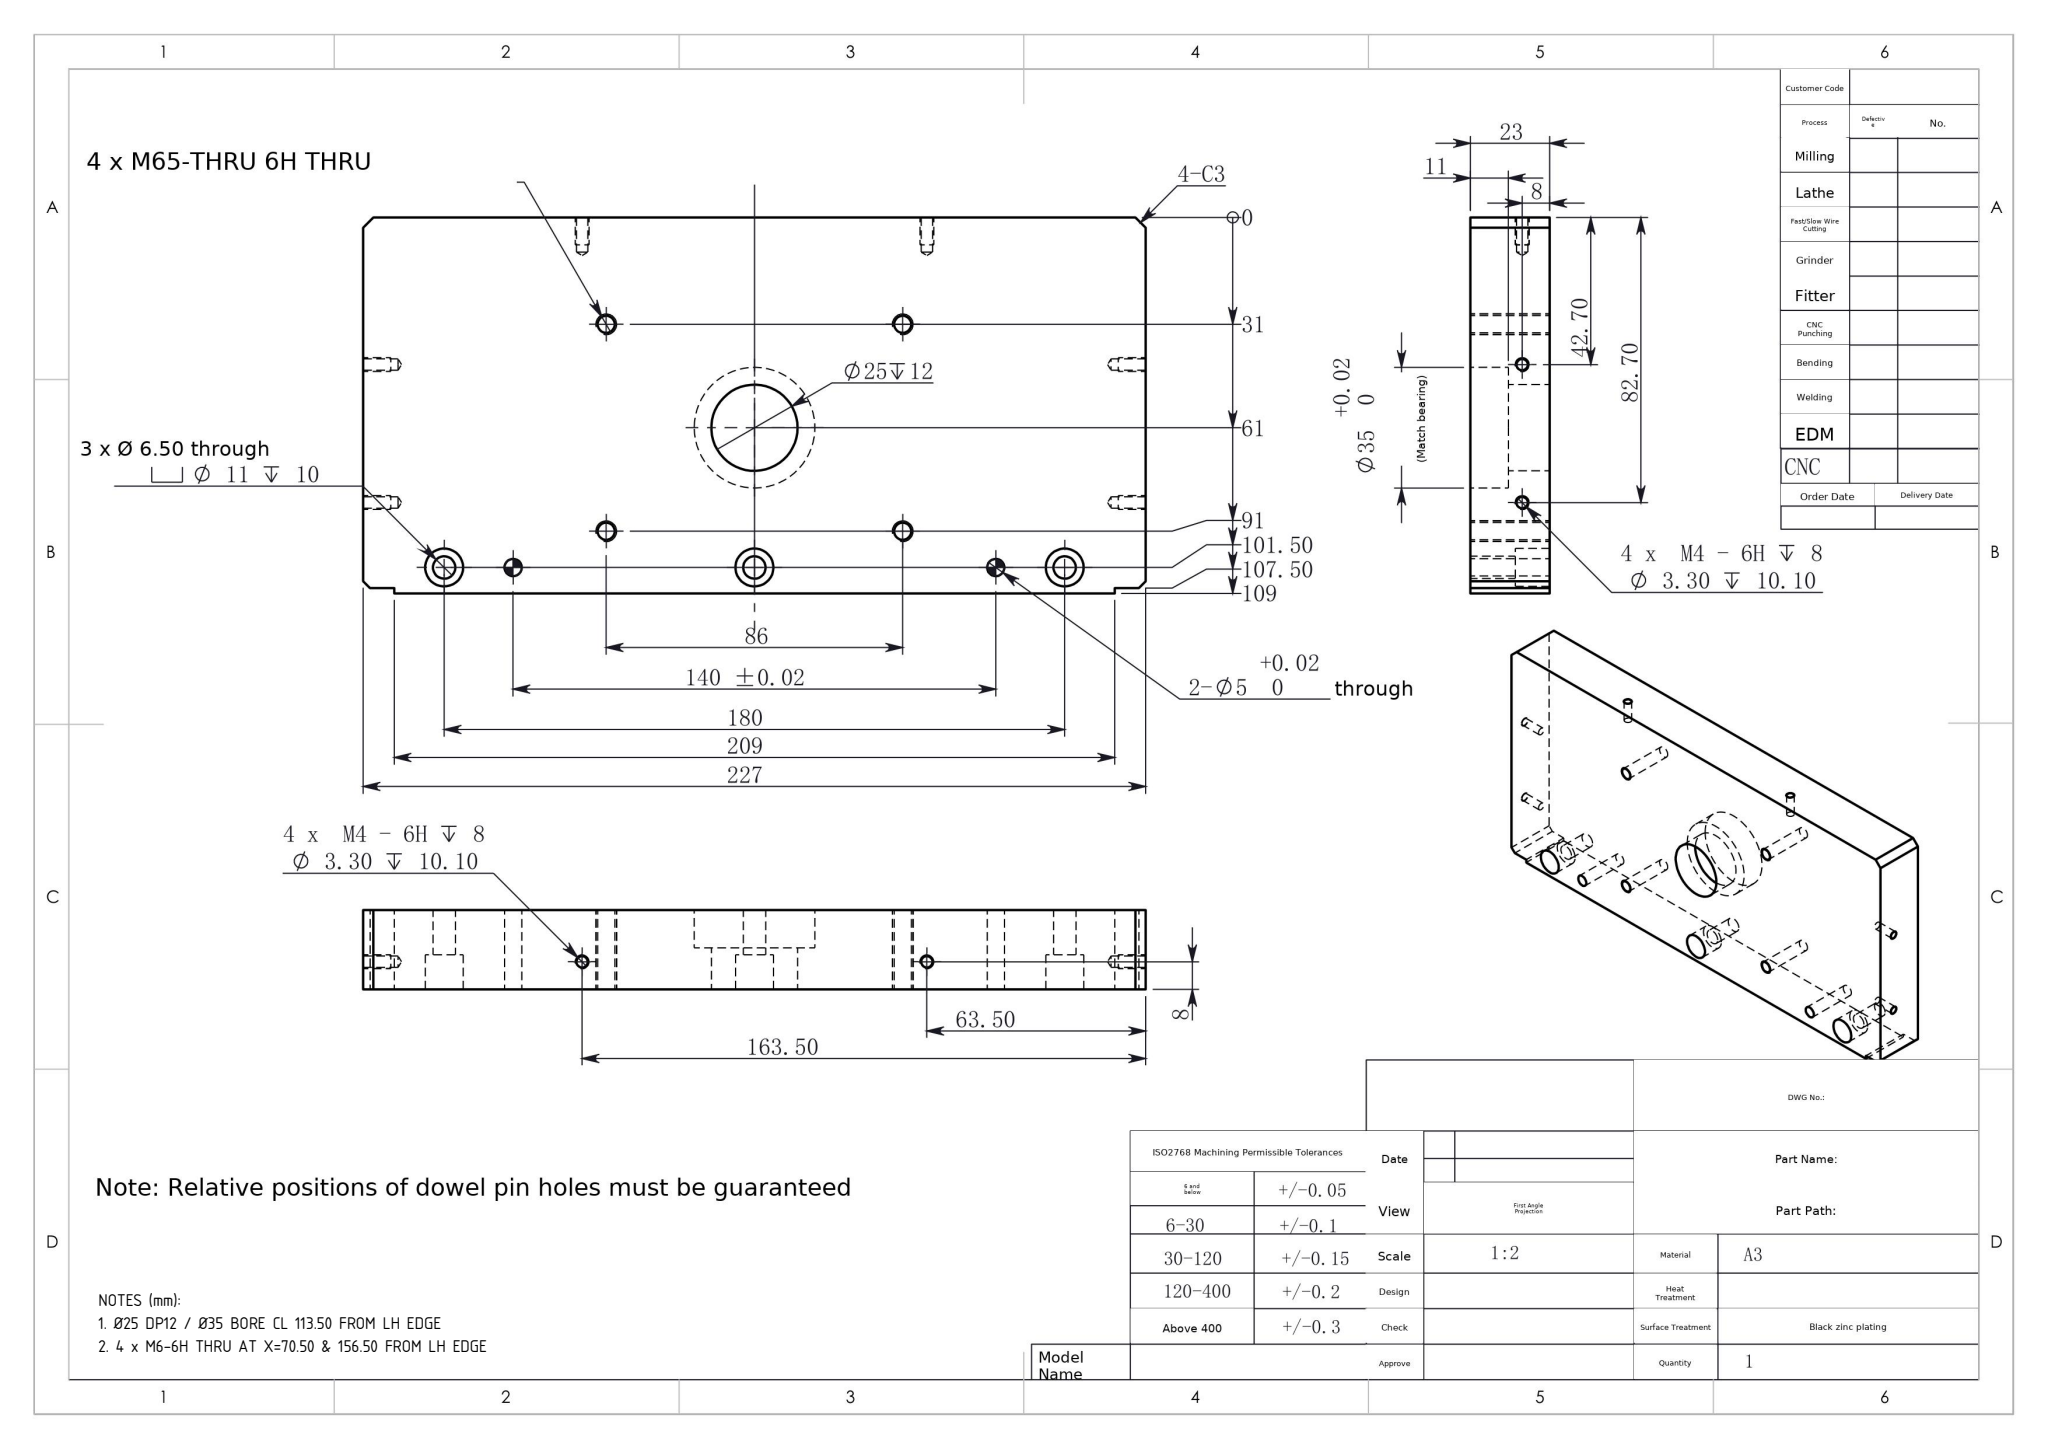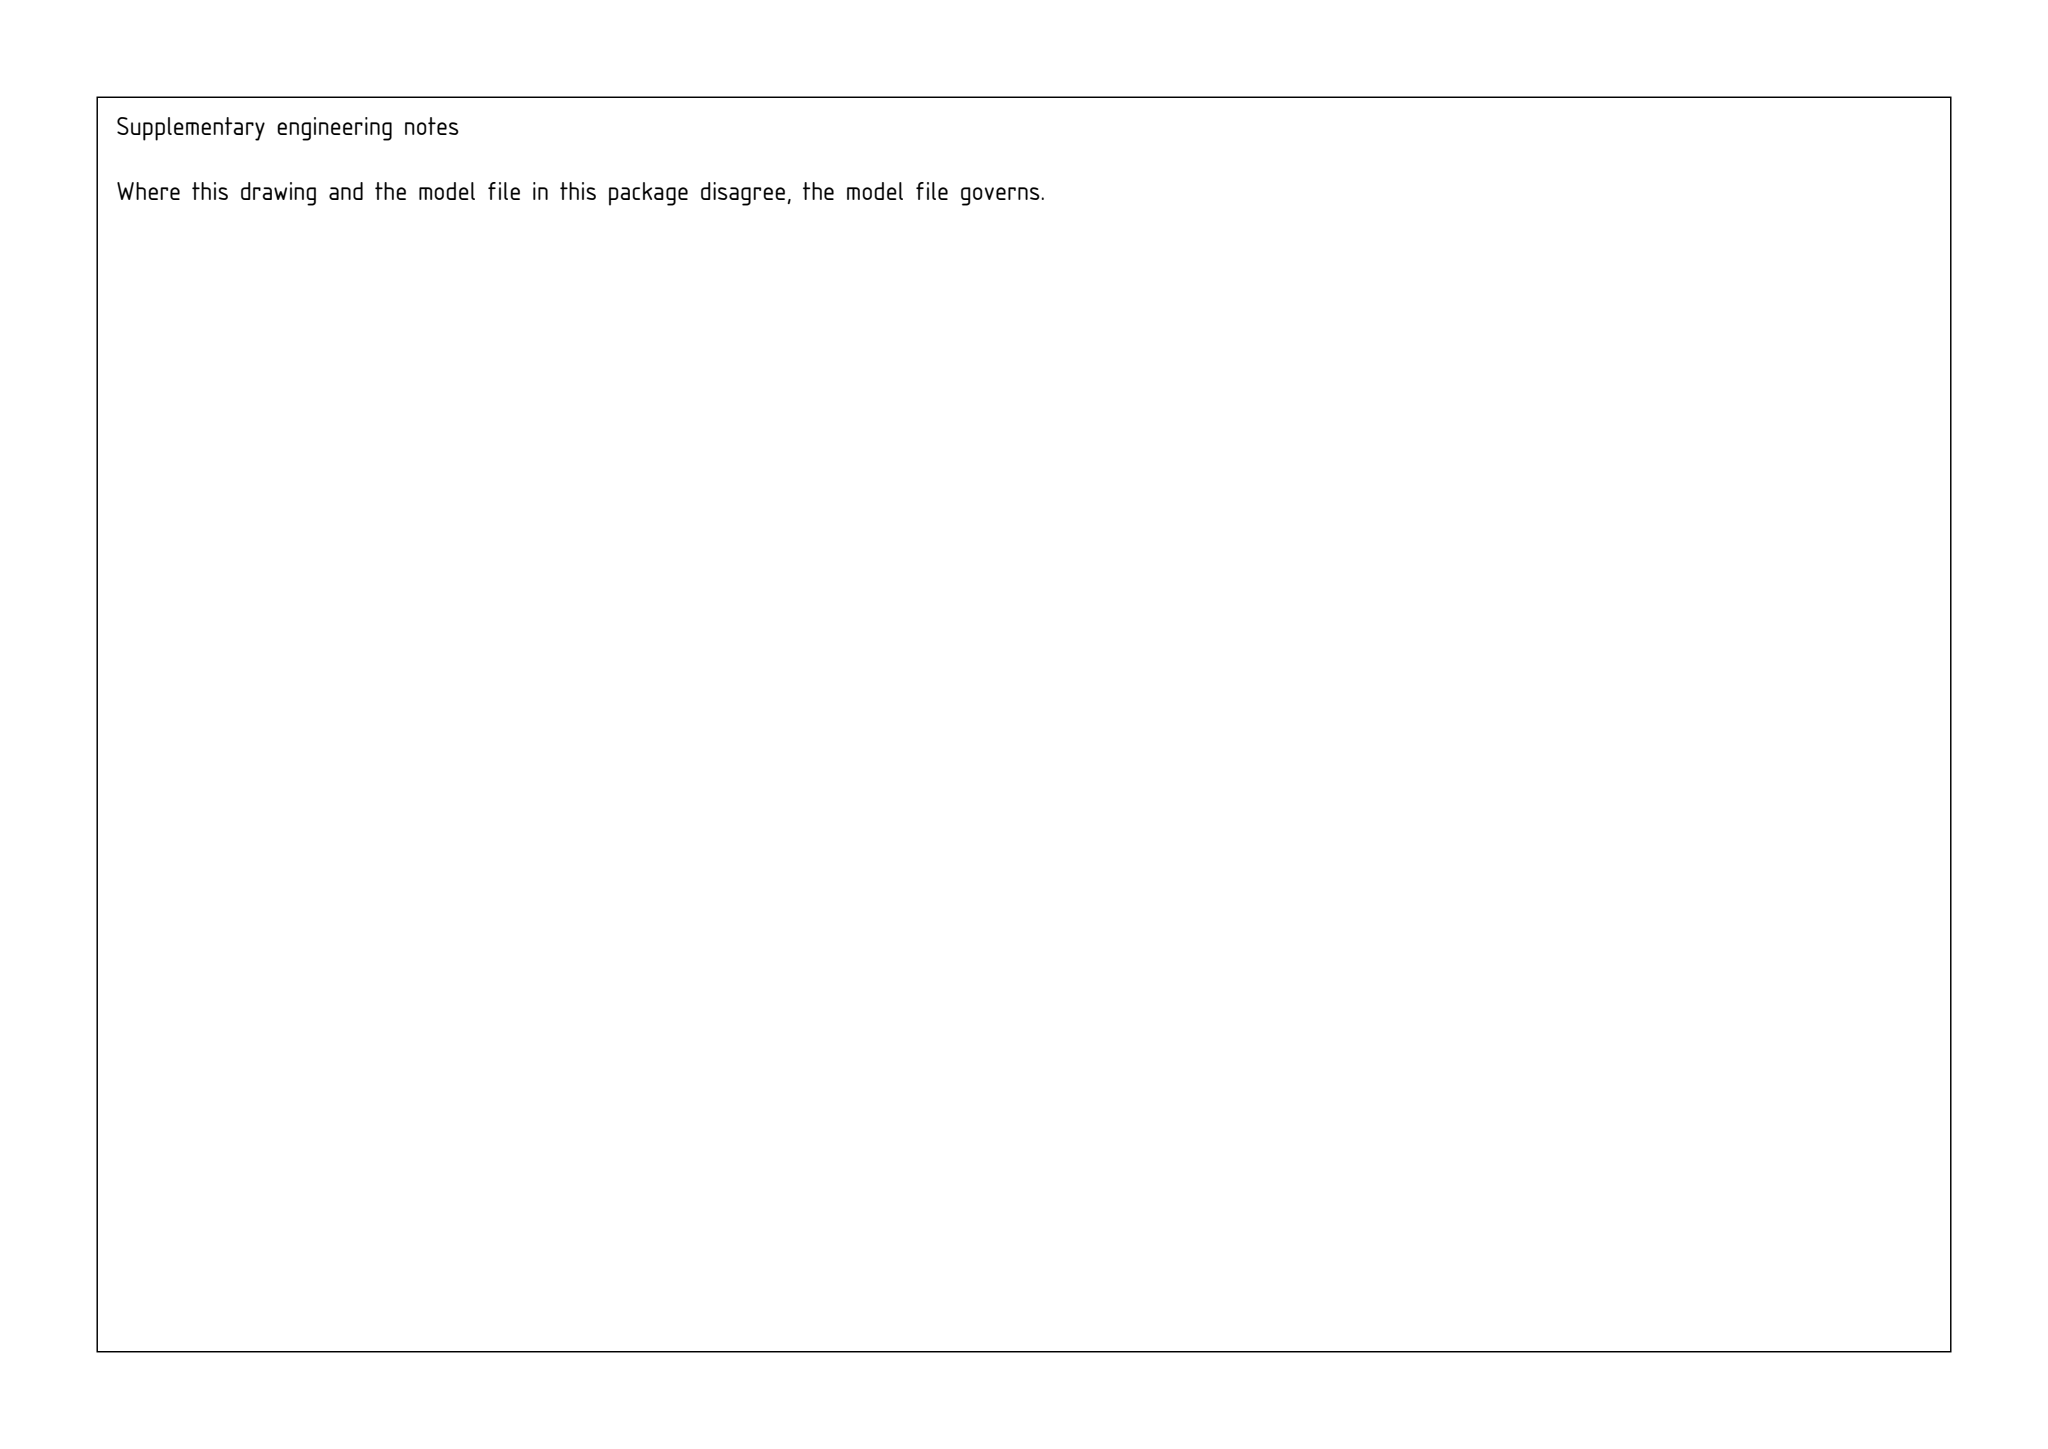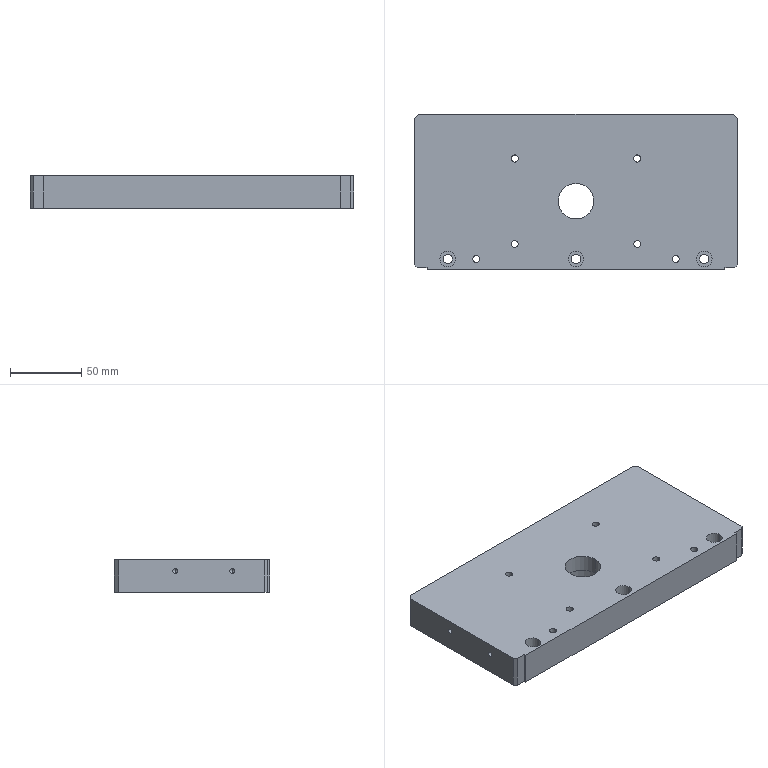Part | SolidWorks | mm | 1 solid | 70 faces | box 227 x 109 x 23 mm | volume 544305 mm3 | cylinder 40 | plane 18 | cone 12 | commonest cylinder face diameters 3.3 x12 5 x12 11 x6 6.5 x6 35 x2 25 x2
Drawing notes:
Ø25 DP12 / Ø35 BORE CL 113.50 FROM LH EDGE | from the solid: Ø25 L12 and Ø35 L11 z-cylinders at (113.5,48.0); bbox X=227, so CL = mid-width
4 x M6-6H THRU AT X=70.50 & 156.50 FROM LH EDGE | from the solid: Ø5.0 z-holes thru 23 at (70.5,18),(70.5,78),(156.5,18),(156.5,78); Ø5 = M6 tap drill
build123d program:
from build123d import *

# Parameters (mm, degrees)
SKETCH4_W                                          = 227
SKETCH4_H                                          = 109
SKETCH4_R                                          = 12.5
SKETCH4_R_2                                        = 2.5
BOSS_EXTRUDE1_DEPTH                                = 23
CHAMFER1_SIZE                                      = 3
HOLE_SIZE_ACCORDING_TO_TYPE_1_OF_HEXAG_D           = 6.5
HOLE_SIZE_ACCORDING_TO_TYPE_1_OF_HEXAG_CBORE_D     = 11
HOLE_SIZE_ACCORDING_TO_TYPE_1_OF_HEXAG_CBORE_DEPTH = 10
M6_TAPPED_HOLE1_D                                  = 5
M4_TAPPED_HOLE2_AT_2_COUNT                         = 2
M4_TAPPED_HOLE2_AT_2_PITCH                         = 40
M4_TAPPED_HOLE3_D                                  = 3.3
M4_TAPPED_HOLE3_DEPTH                              = 10.1
M4_TAPPED_HOLE3_TIP                                = 0.9914
SKETCH17_W                                         = 9
SKETCH17_H                                         = 1.5
CUT_EXTRUDE2_DEPTH                                 = 128.99
CHAMFER2_SIZE                                      = 2
SKETCH10_R                                         = 17.5
CUT_EXTRUDE3_DEPTH                                 = 11


with BuildPart() as part:
    # Sketch4 → Boss-Extrude1 (new body)
    with BuildSketch(Plane.XY):
        Rectangle(SKETCH4_W, SKETCH4_H)
        with Locations((0, -6.5)):
            Circle(SKETCH4_R, mode=Mode.SUBTRACT)
        with Locations((-70, -47)):
            Circle(SKETCH4_R_2, mode=Mode.SUBTRACT)
        with Locations(Location((70, -47, 0), (0, 0, 180))):
            Circle(SKETCH4_R_2, mode=Mode.SUBTRACT)
    extrude(amount=BOSS_EXTRUDE1_DEPTH)

    # Chamfer1
    chamfer1_edges = [part.edges().sort_by_distance(p)[0] for p in [
        (-113.5, 54.5, 11.5),
        (113.5, 54.5, 11.5),
    ]]
    chamfer(chamfer1_edges, length=CHAMFER1_SIZE)

    # Hole Size _According to_ Type 1 of Hexag (through all)
    with Locations(Plane.XY.offset(23)):
        with Locations((90, -47), (-90, -47), (0, -47)):
            CounterBoreHole(HOLE_SIZE_ACCORDING_TO_TYPE_1_OF_HEXAG_D / 2, HOLE_SIZE_ACCORDING_TO_TYPE_1_OF_HEXAG_CBORE_D / 2, HOLE_SIZE_ACCORDING_TO_TYPE_1_OF_HEXAG_CBORE_DEPTH)

    # M6 Tapped Hole1 (through all)
    with Locations(Plane.XY.offset(23)):
        with Locations((-43, -36.5), (-43, 23.5), (43, 23.5), (43, -36.5)):
            Hole(M6_TAPPED_HOLE1_D / 2)

    # Sketch14 → M4 Tapped Hole2 (revolve, cut)
    with BuildSketch(Plane(origin=(-113.5, -28.2, 15), x_dir=(0, 0, 1), z_dir=(0, 1, 0))):
        Polygon((0, 0), (0, 11.091), (1.65, 10.1), (1.65, 0), align=None)
    m4_tapped_hole2 = revolve(axis=Axis((-119.85, -28.2, 15), (1, 0, 0)), mode=Mode.SUBTRACT)

    # M4 Tapped Hole2 at 2: M4 Tapped Hole2 ×2
    with Locations(*[(0, i * M4_TAPPED_HOLE2_AT_2_PITCH, 0) for i in range(1, M4_TAPPED_HOLE2_AT_2_COUNT)]):
        add(m4_tapped_hole2, mode=Mode.SUBTRACT)

    # M4 Tapped Hole3
    with Locations(Plane(origin=(0, 54.5, 0), x_dir=(1, 0, 0), z_dir=(0, 1, 0))):
        with Locations((50, -15), (-50, -15)):
            Hole(M4_TAPPED_HOLE3_D / 2, depth=M4_TAPPED_HOLE3_DEPTH)
            with Locations((0, 0, -(M4_TAPPED_HOLE3_DEPTH + M4_TAPPED_HOLE3_TIP / 2))):  # 118° drill point
                Cone(0, M4_TAPPED_HOLE3_D / 2, M4_TAPPED_HOLE3_TIP, mode=Mode.SUBTRACT)

    # Sketch17 → Cut-Extrude2 (cut, through all)
    with BuildSketch(Plane(origin=(0, 0, 0), x_dir=(-1, 0, 0), z_dir=(0, 0, -1))):
        with Locations((-109, -53.75)):
            Rectangle(SKETCH17_W, SKETCH17_H)
        with Locations((109, -53.75)):
            Rectangle(SKETCH17_W, SKETCH17_H)
    extrude(amount=-CUT_EXTRUDE2_DEPTH, mode=Mode.SUBTRACT)

    # Chamfer2
    chamfer2_edges = [part.edges().sort_by_distance(p)[0] for p in [
        (113.5, -53, 11.5),
        (-113.5, -53, 11.5),
    ]]
    chamfer(chamfer2_edges, length=CHAMFER2_SIZE)

    # Sketch10 → Cut-Extrude3 (cut)
    with BuildSketch(Plane(origin=(0, 0, 0), x_dir=(-1, 0, 0), z_dir=(0, 0, -1))):
        with Locations((0, -6.5)):
            Circle(SKETCH10_R)
    extrude(amount=-CUT_EXTRUDE3_DEPTH, mode=Mode.SUBTRACT)

    # Mirror1: M4 Tapped Hole2 across plane
    add(m4_tapped_hole2.mirror(Plane(origin=(0, 0, 0), x_dir=(0, 0, 1), z_dir=(1, 0, 0))), mode=Mode.SUBTRACT)

    # Mirror1 copy 1 sketch → Mirror1 copy 1 (revolve, cut)
    with BuildSketch(Plane(origin=(113.5, 11.8, 15), x_dir=(0, 0, 1), z_dir=(0, 1, 0))):
        Polygon((0, 0), (0, -11.091), (1.65, -10.1), (1.65, 0), align=None)
    revolve(axis=Axis((119.85, 11.8, 15), (1, 0, 0)), mode=Mode.SUBTRACT)


solid = part.part